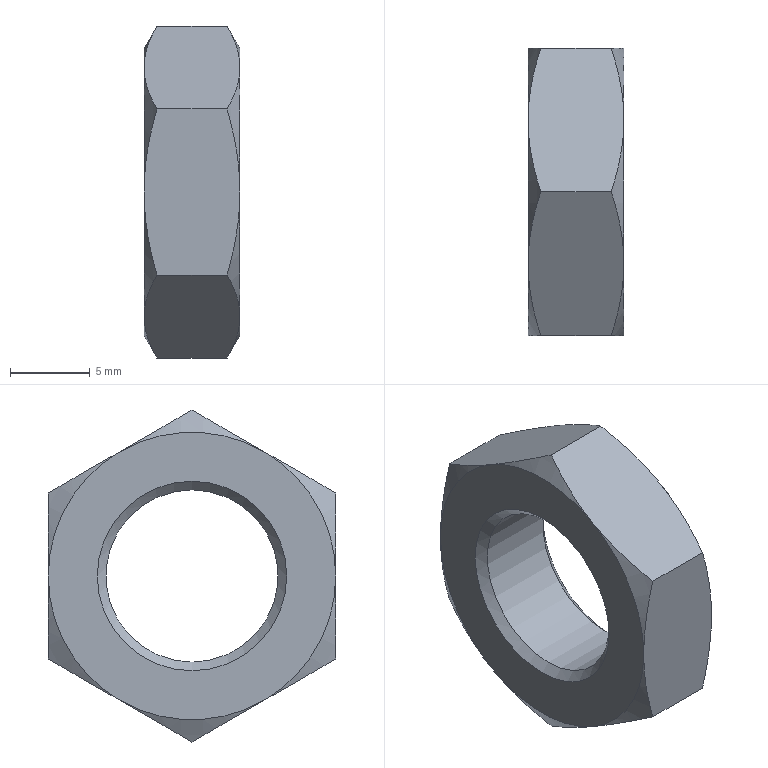Component | NX | GB-T6173-2000_M12X1_5 | 1 solid | 23 faces | volume 1113 mm3 | cone 14 | plane 8 | cylinder 1 | commonest cylinder face diameters 10.782 x1